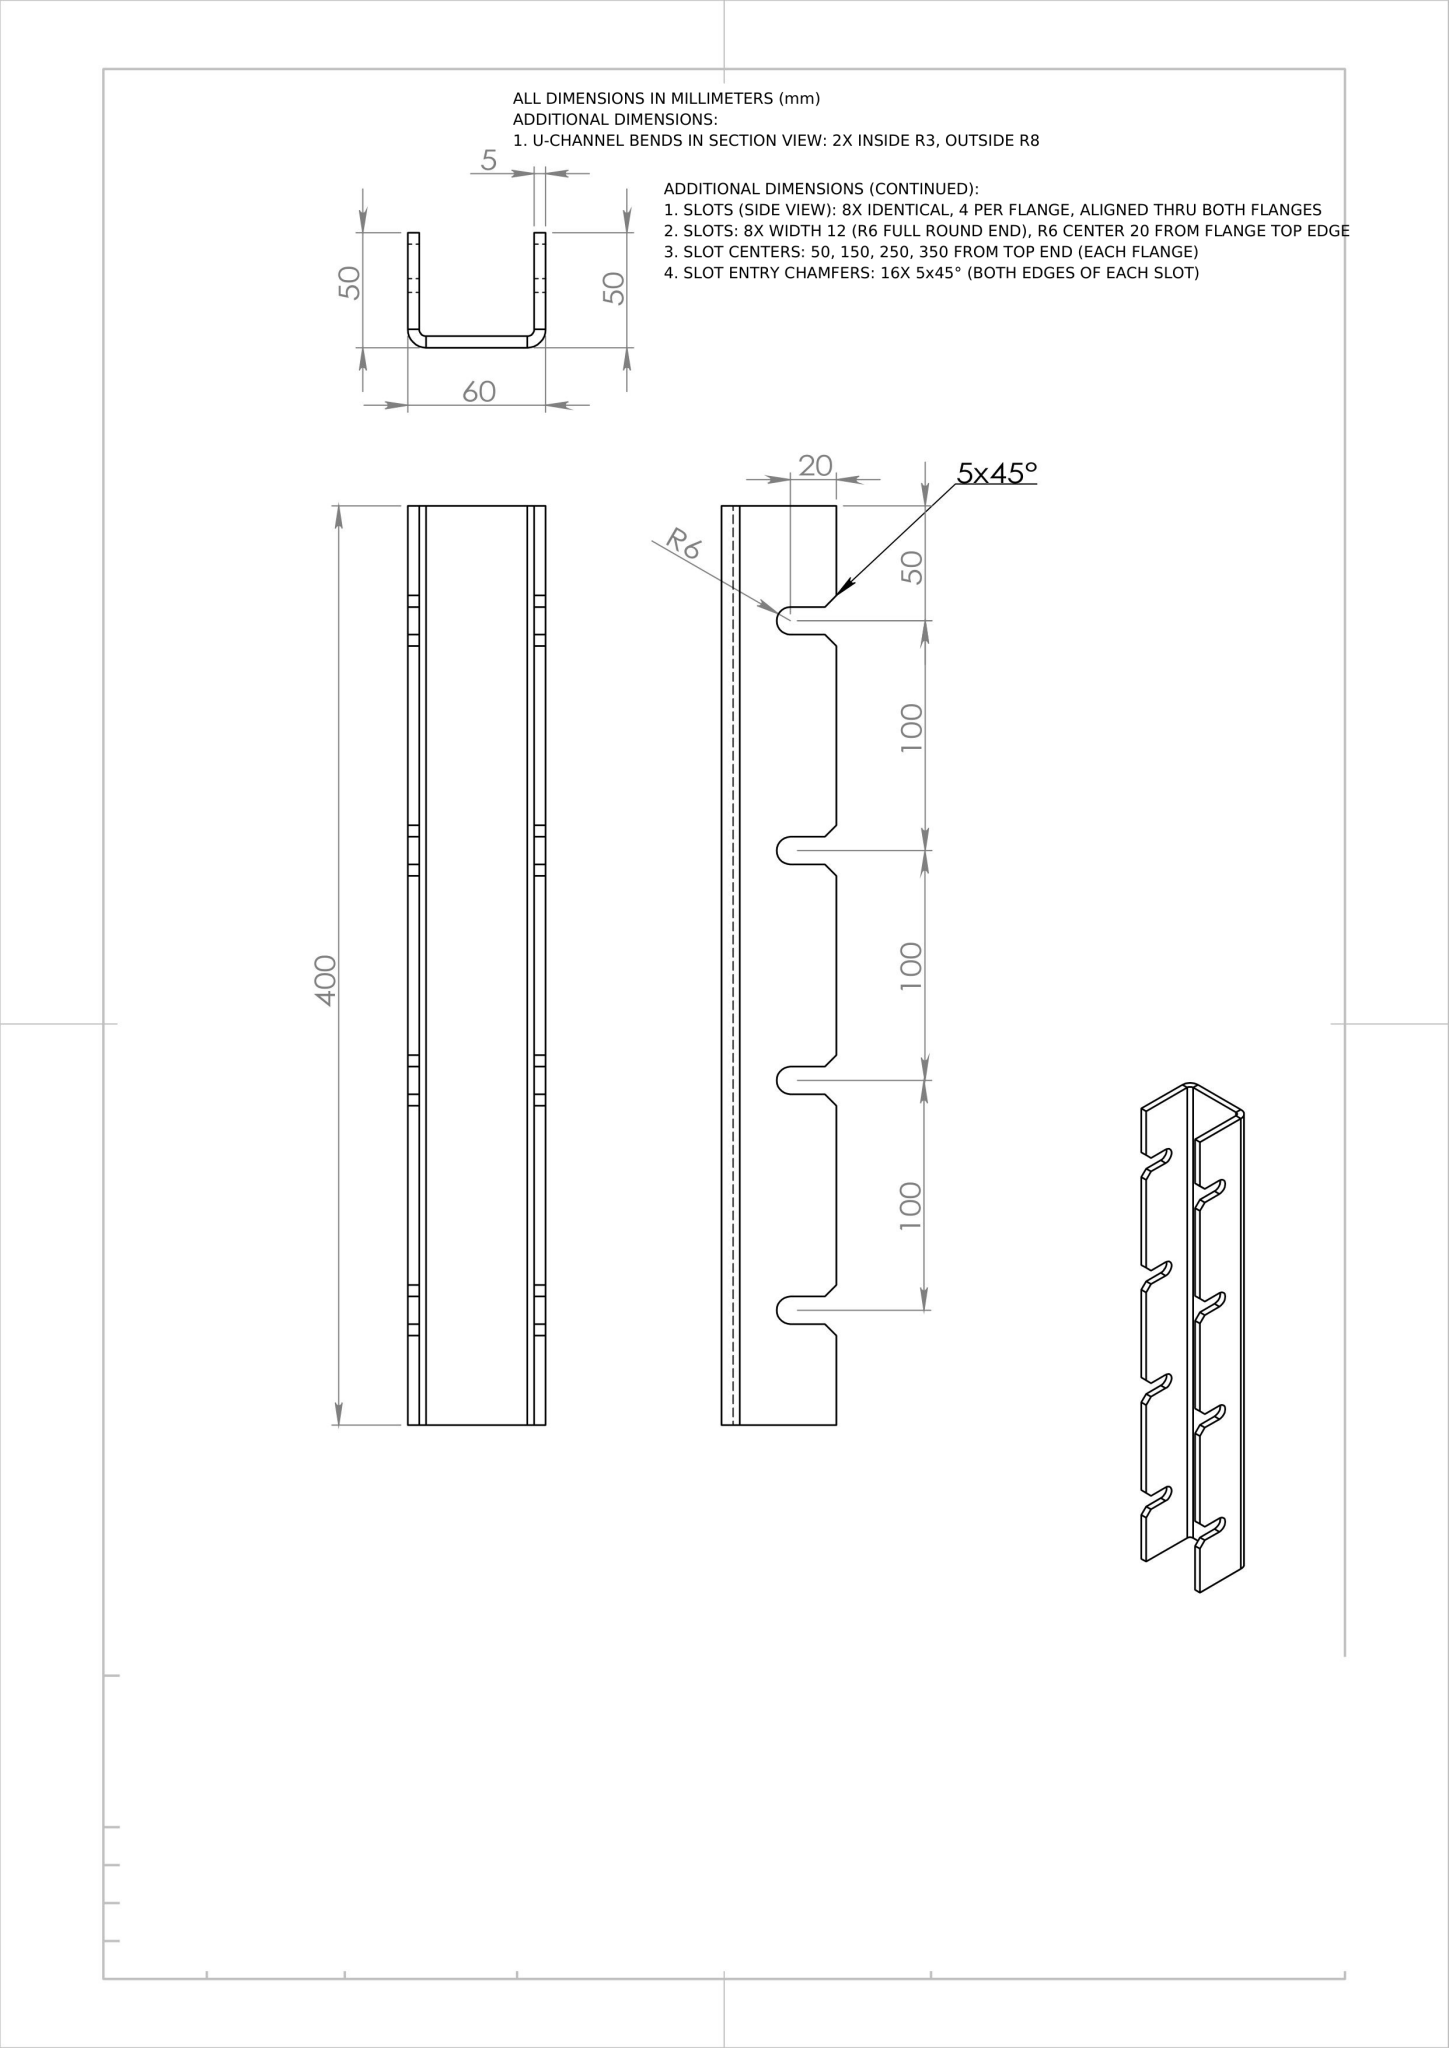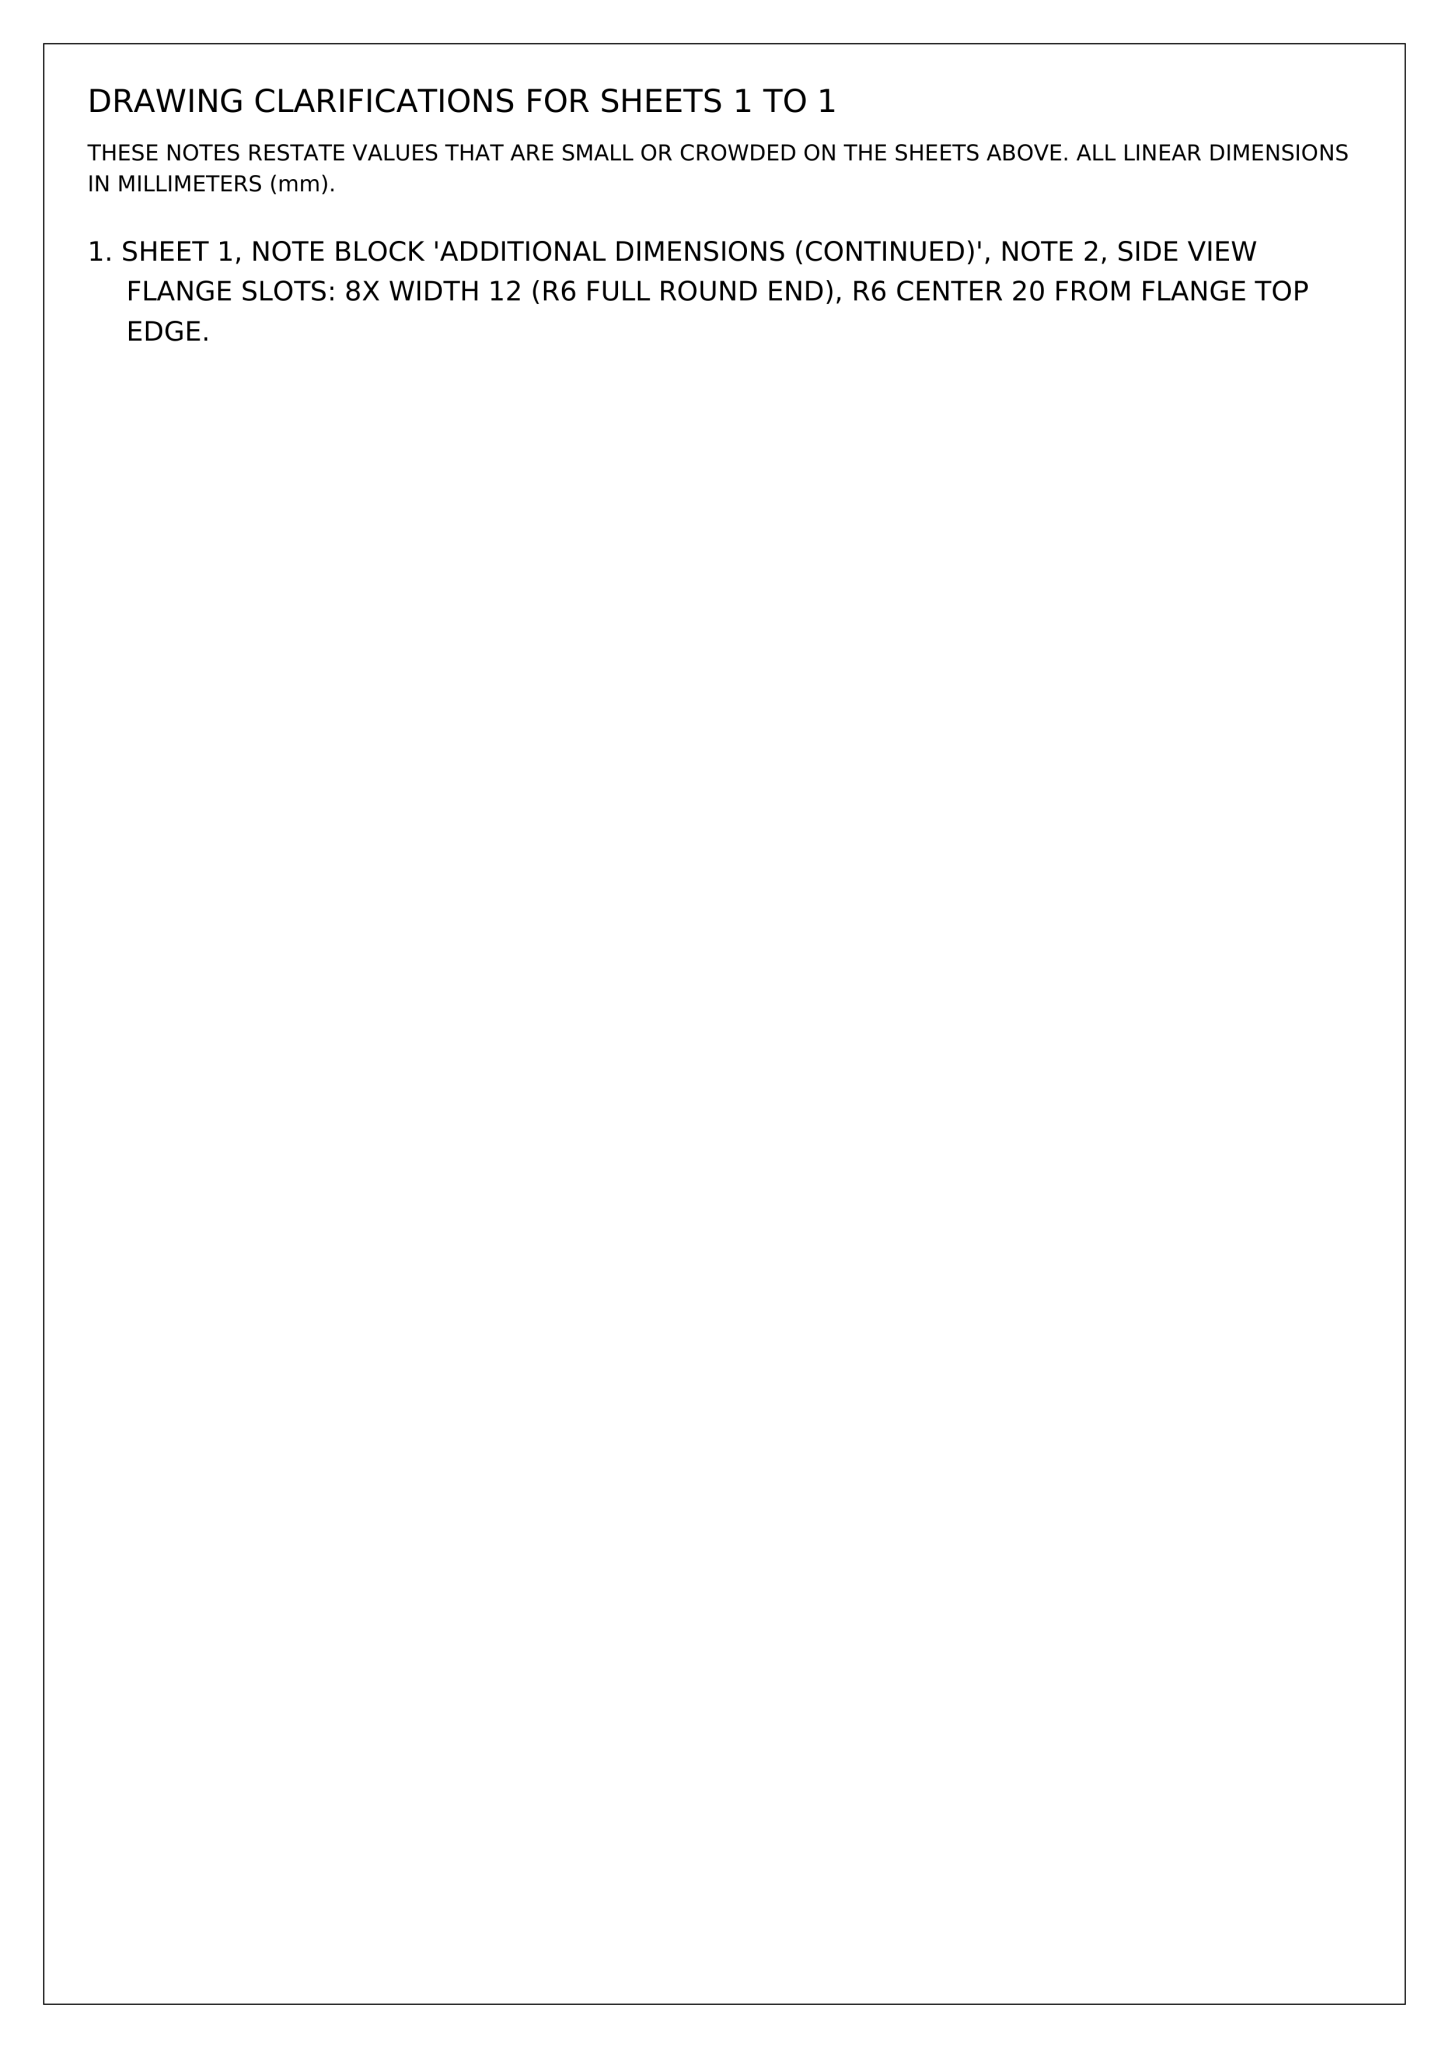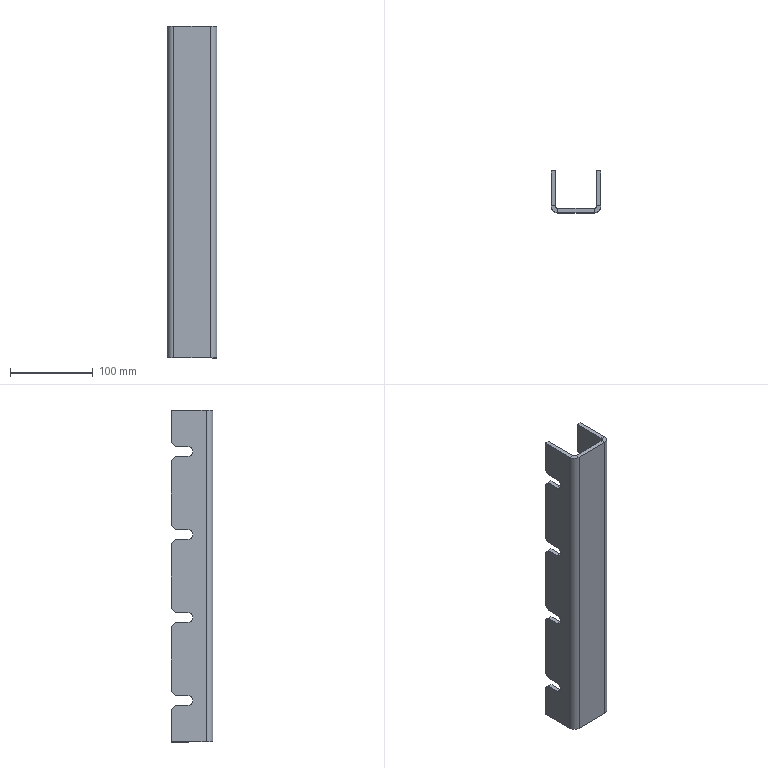Part | NX | mm | 1 solid | 70 faces | box 60 x 50 x 400 mm | volume 277696 mm3 | plane 58 | cylinder 12 | commonest cylinder face diameters 12 x8 16 x2 6 x2